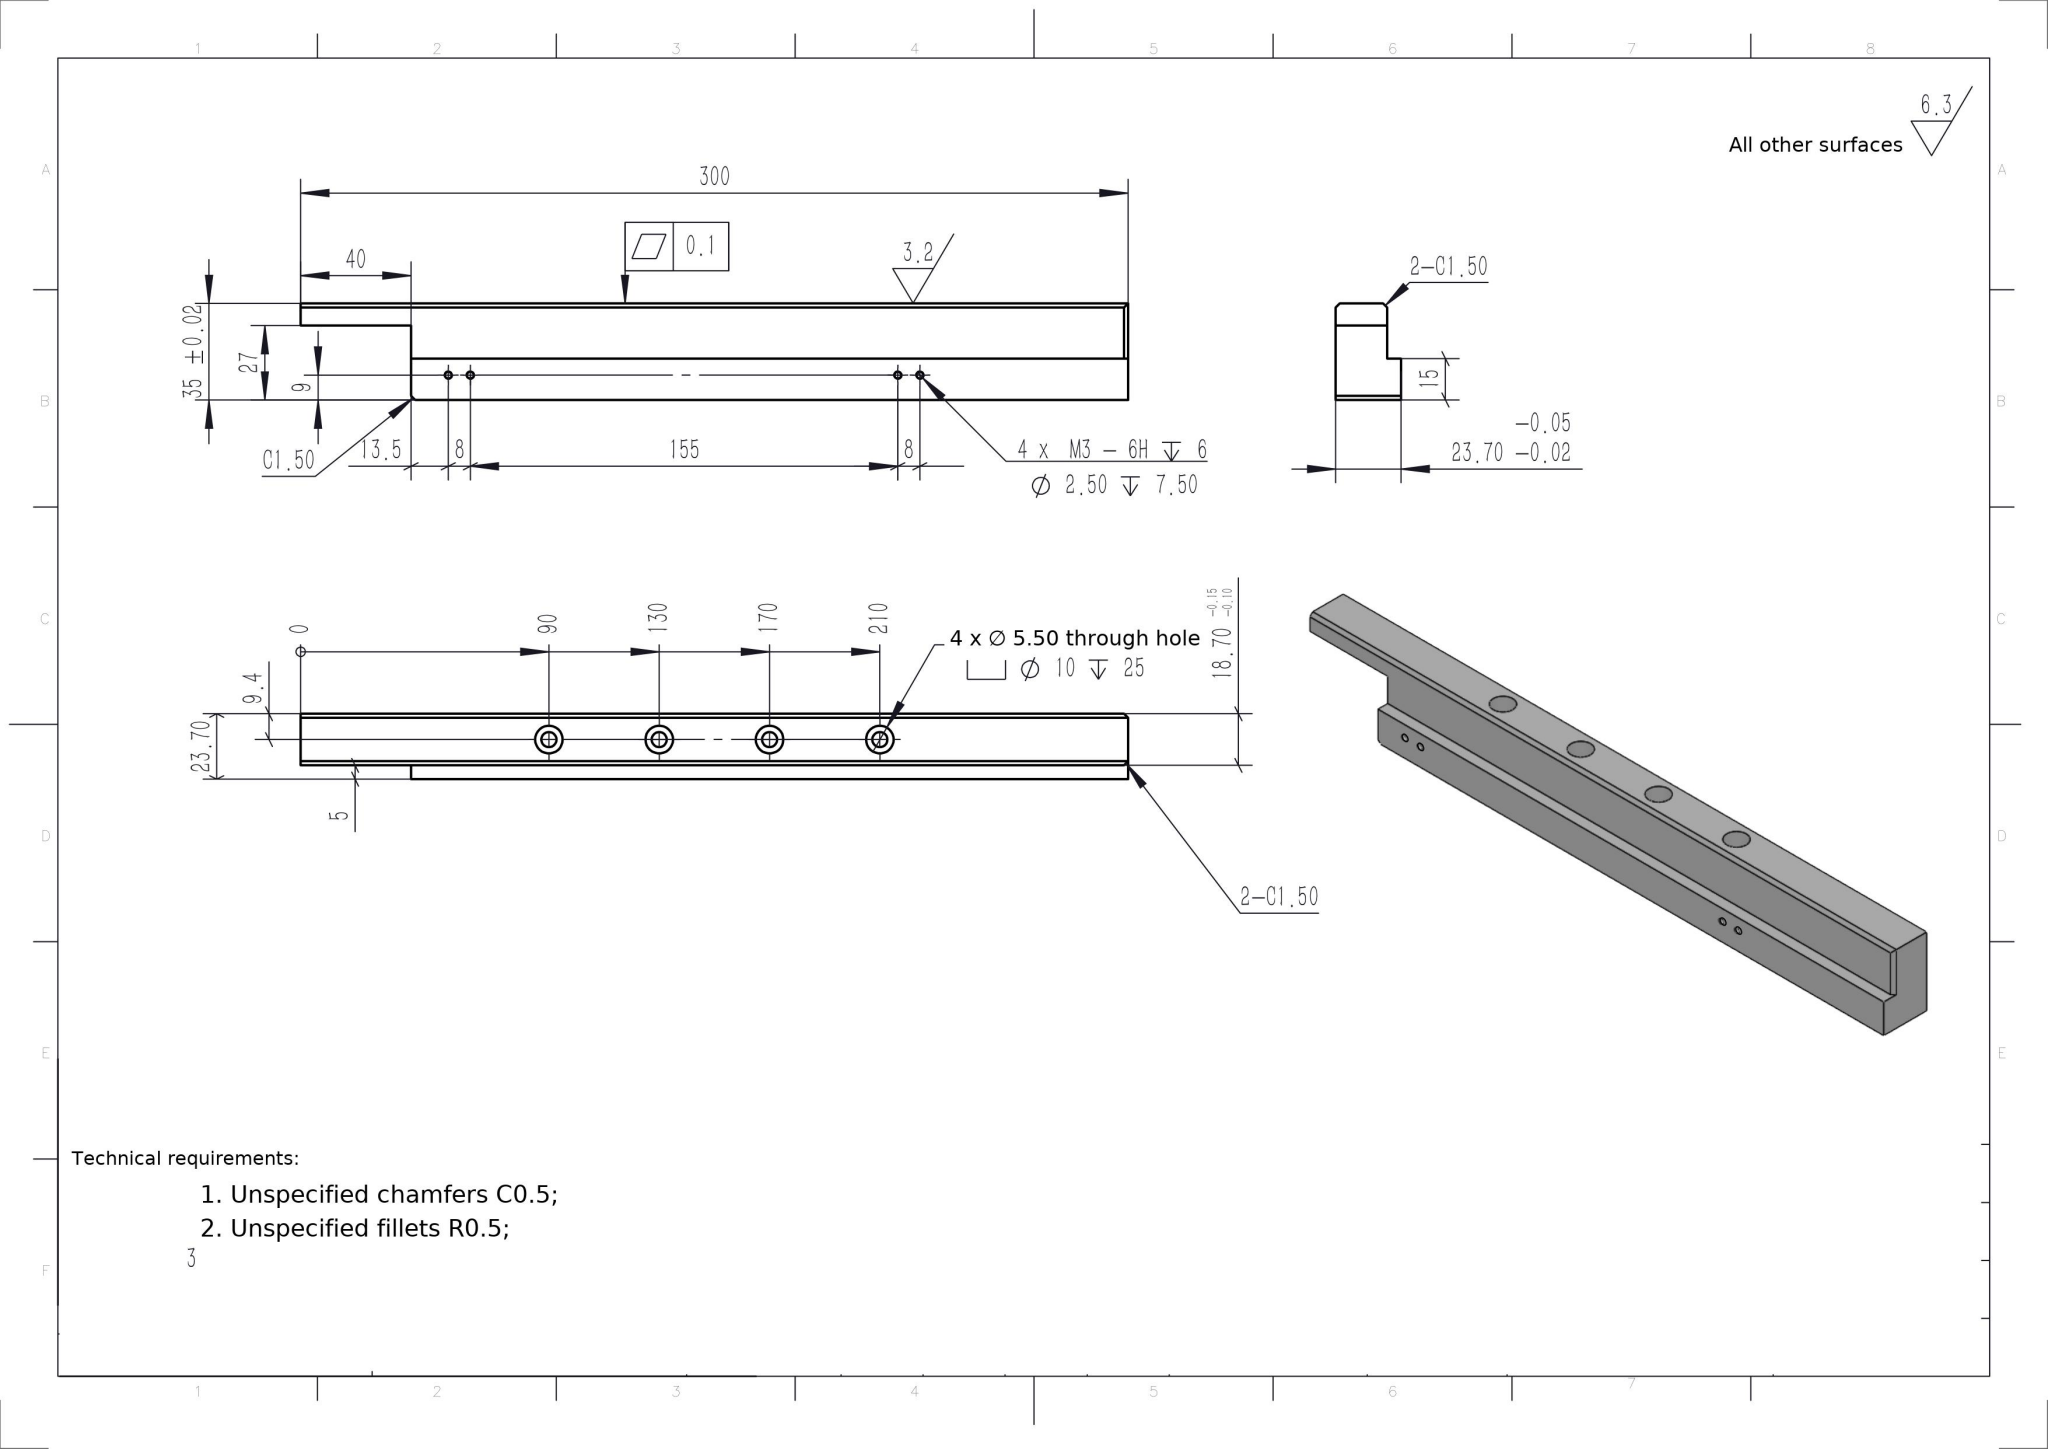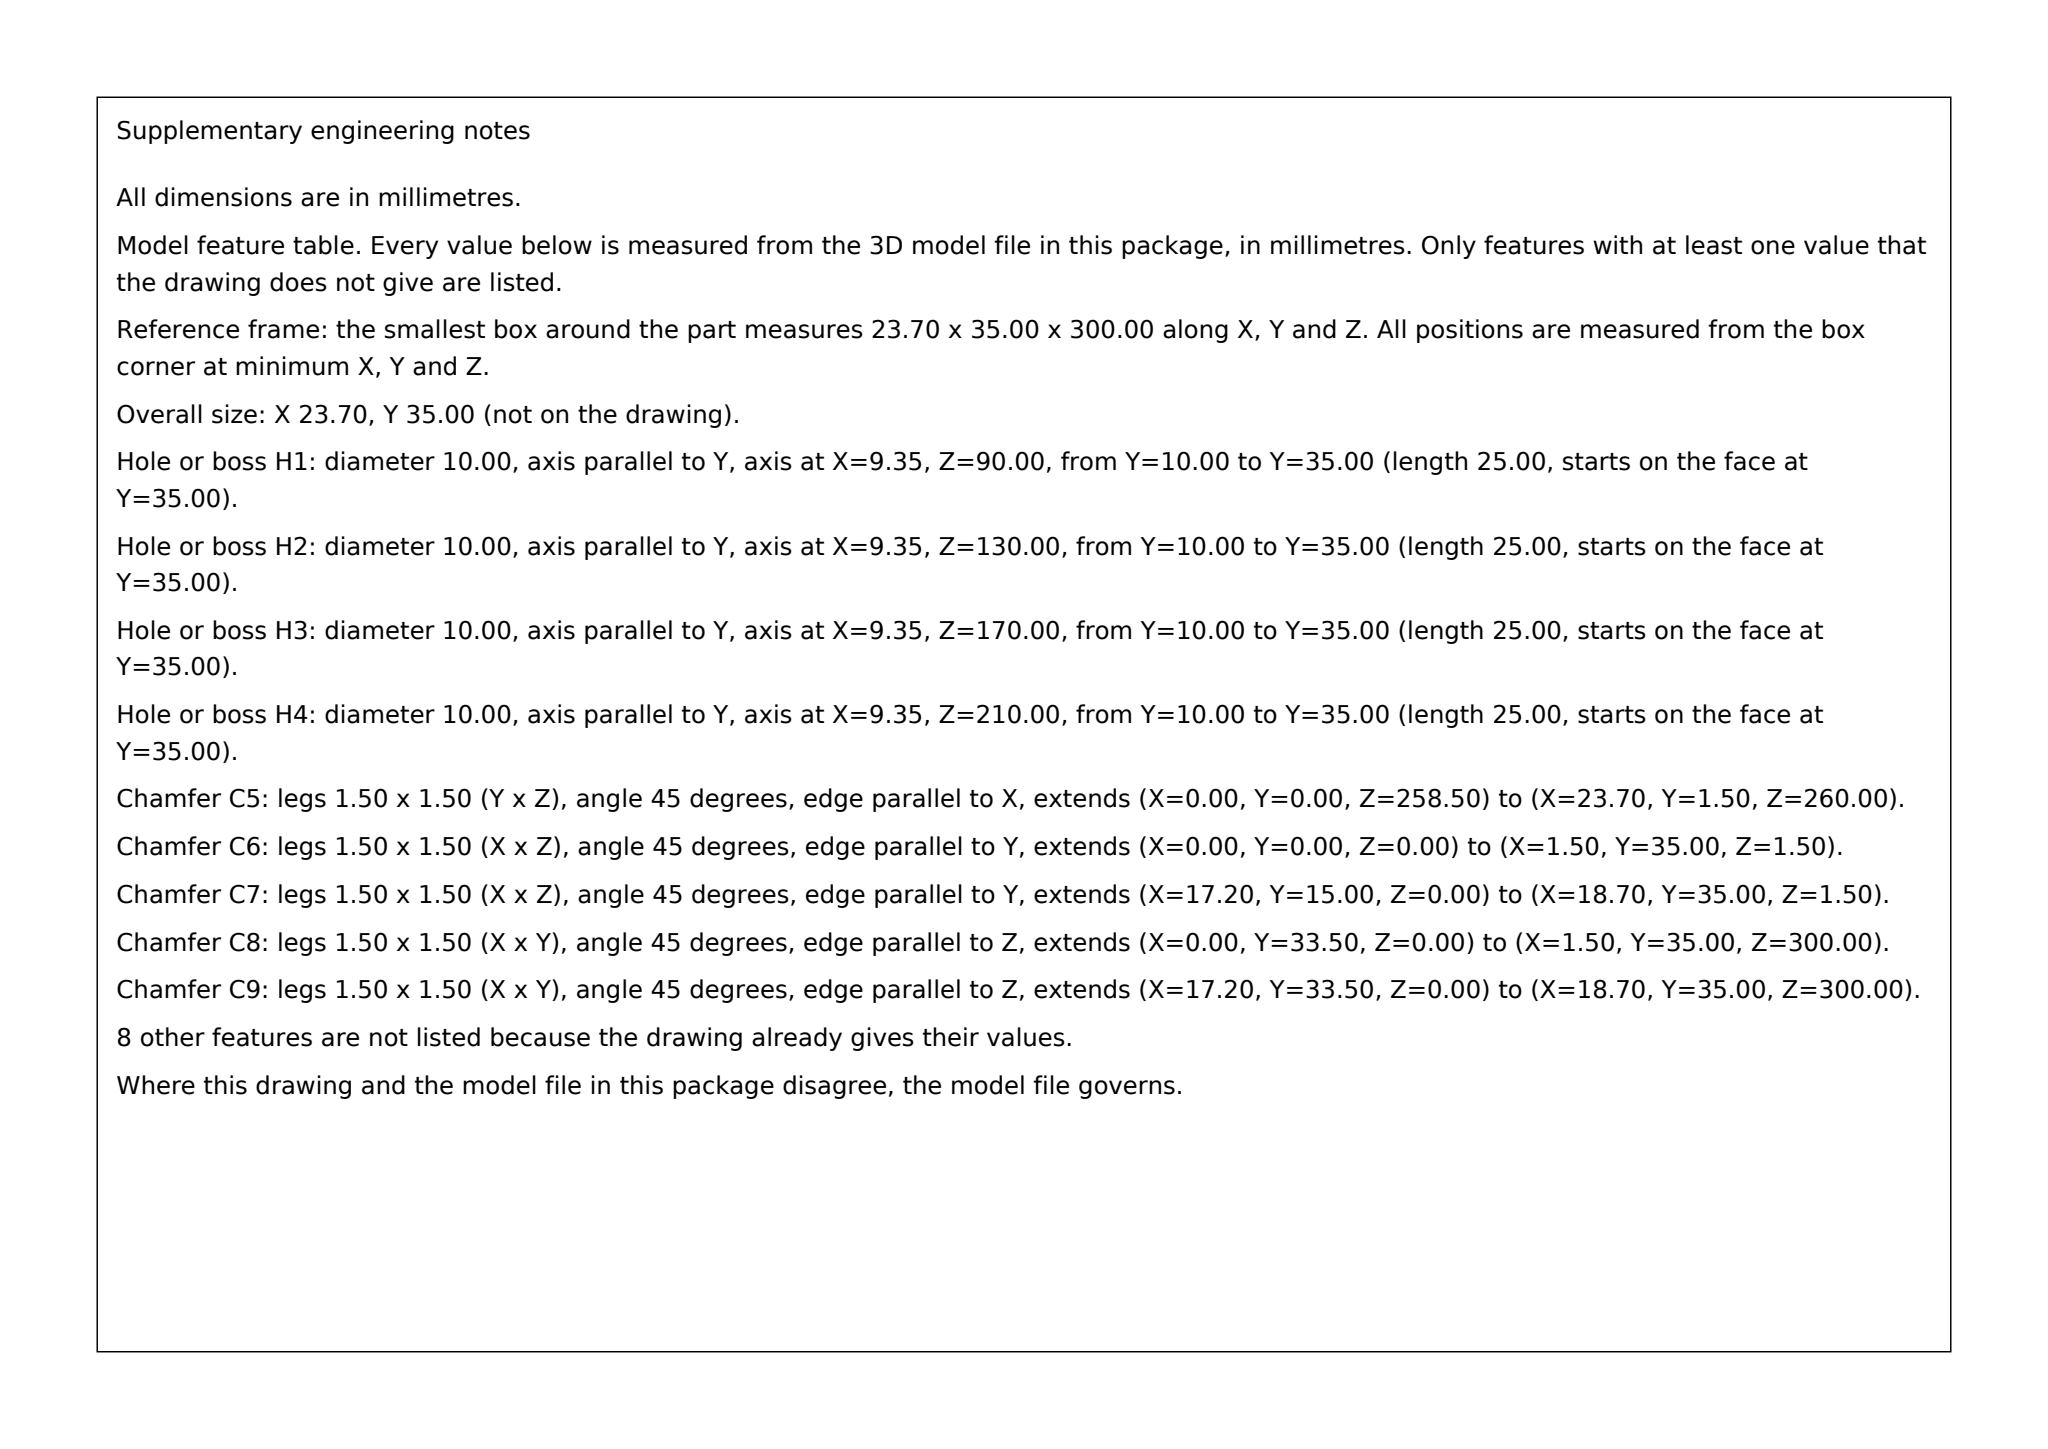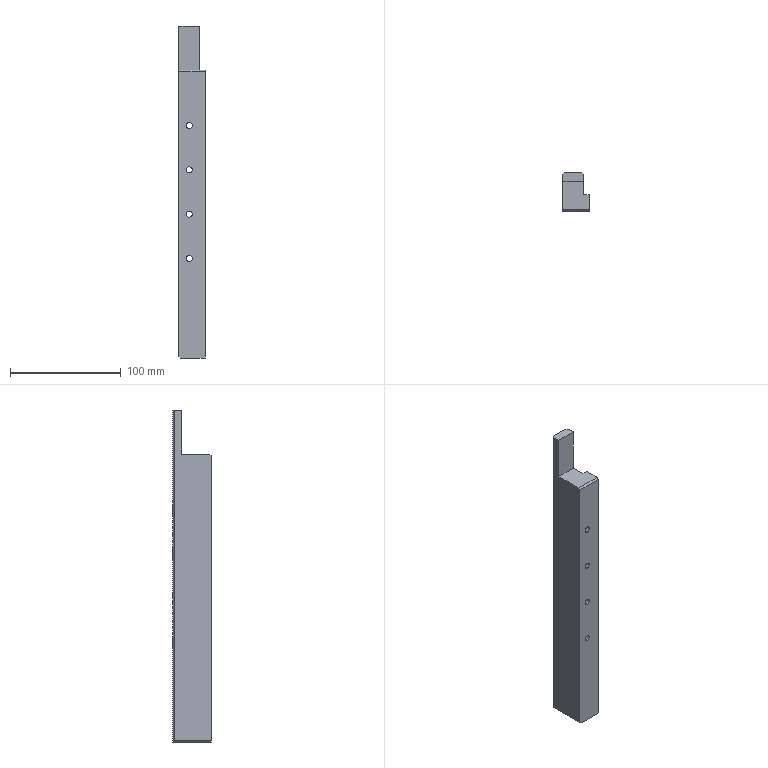Part | SolidWorks | mm | 1 solid | 51 faces | box 23.7 x 35 x 300 mm | volume 185936 mm3 | cylinder 24 | plane 19 | cone 8 | commonest cylinder face diameters 2.5 x8 10 x8 5.5 x8
build123d program:
from build123d import *

# Parameters (mm, degrees)
BOSS_EXTRUDE1_DEPTH                               = 300
HOLE_SIZE_ACCORDING_TO_HEXAGON_SOCKET_D           = 5.5
HOLE_SIZE_ACCORDING_TO_HEXAGON_SOCKET_CBORE_D     = 10
HOLE_SIZE_ACCORDING_TO_HEXAGON_SOCKET_CBORE_DEPTH = 25
SKETCH10_W                                        = 300
SKETCH10_H                                        = 15
BOSS_EXTRUDE2_DEPTH                               = 5
M3_TAPPED_HOLE1_D                                 = 2.5
M3_TAPPED_HOLE1_DEPTH                             = 7.5
M3_TAPPED_HOLE1_TIP                               = 0.7511
SKETCH13_W                                        = 40
SKETCH13_H                                        = 15
CUT_EXTRUDE1_DEPTH                                = 303.963
CHAMFER1_SIZE                                     = 1.5
SKETCH16_W                                        = 40
SKETCH16_H                                        = 12
CUT_EXTRUDE2_DEPTH                                = 303.613


with BuildPart() as part:
    # Sketch1 → Boss-Extrude1 (new body)
    with BuildSketch(Plane.XY):
        Polygon((-9.35, 0), (9.35, 0), (9.35, 35), (-6.265, 35), (-9.35, 35), align=None)
    extrude(amount=BOSS_EXTRUDE1_DEPTH)

    # Hole Size _ according to_ Hexagon Socket (through all)
    with Locations(Plane(origin=(0, 35, 0), x_dir=(1, 0, 0), z_dir=(0, 1, 0))):
        with Locations((0, -90), (0, -130), (0, -170), (0, -210)):
            CounterBoreHole(HOLE_SIZE_ACCORDING_TO_HEXAGON_SOCKET_D / 2, HOLE_SIZE_ACCORDING_TO_HEXAGON_SOCKET_CBORE_D / 2, HOLE_SIZE_ACCORDING_TO_HEXAGON_SOCKET_CBORE_DEPTH)

    # Sketch10 → Boss-Extrude2 (add)
    with BuildSketch(Plane(origin=(9.35, 0, 0), x_dir=(0, 0, -1), z_dir=(1, 0, 0))):
        with Locations((-150, 7.5)):
            Rectangle(SKETCH10_W, SKETCH10_H)
    extrude(amount=BOSS_EXTRUDE2_DEPTH)

    # M3 Tapped Hole1
    with Locations(Plane(origin=(14.35, 0, 0), x_dir=(0, 0, -1), z_dir=(1, 0, 0))):
        with Locations((-238.5, 9), (-246.5, 9), (-83.5, 9), (-75.5, 9)):
            Hole(M3_TAPPED_HOLE1_D / 2, depth=M3_TAPPED_HOLE1_DEPTH)
            with Locations((0, 0, -(M3_TAPPED_HOLE1_DEPTH + M3_TAPPED_HOLE1_TIP / 2))):  # 118° drill point
                Cone(0, M3_TAPPED_HOLE1_D / 2, M3_TAPPED_HOLE1_TIP, mode=Mode.SUBTRACT)

    # Sketch13 → Cut-Extrude1 (cut, through all)
    with BuildSketch(Plane(origin=(14.35, 0, 0), x_dir=(0, 0, -1), z_dir=(1, 0, 0))):
        with Locations((-280, 7.5)):
            Rectangle(SKETCH13_W, SKETCH13_H)
    extrude(amount=-CUT_EXTRUDE1_DEPTH, mode=Mode.SUBTRACT)

    # Chamfer1
    chamfer1_edges = [part.edges().sort_by_distance(p)[0] for p in [
        (2.5, 0, 260),
        (-9.35, 17.5, 0),
        (9.35, 25, 0),
        (-9.35, 35, 150),
        (9.35, 35, 150),
    ]]
    chamfer(chamfer1_edges, length=CHAMFER1_SIZE)

    # Sketch16 → Cut-Extrude2 (cut, through all)
    with BuildSketch(Plane(origin=(9.35, 0, 0), x_dir=(0, 0, -1), z_dir=(1, 0, 0))):
        with Locations((-280, 21)):
            Rectangle(SKETCH16_W, SKETCH16_H)
    extrude(amount=-CUT_EXTRUDE2_DEPTH, mode=Mode.SUBTRACT)


solid = part.part